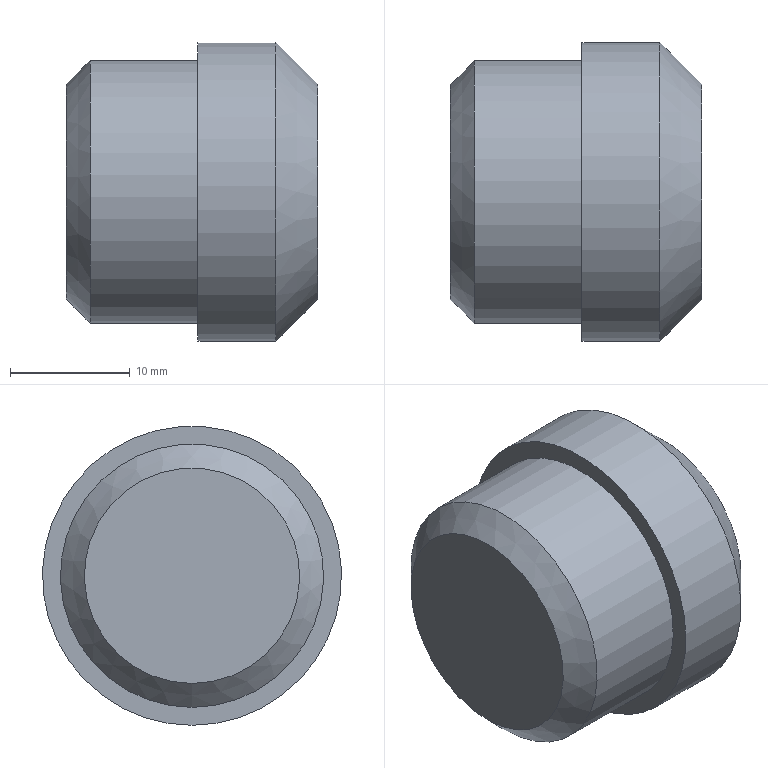Component | NX | TOP_BLOCK | 1 solid | 7 faces | box 21 x 25 x 25 mm | volume 8524 mm3 | plane 3 | cone 2 | cylinder 2 | commonest cylinder face diameters 25 x1 22 x1
STEP:
#1=CARTESIAN_POINT('',(0.,0.,0.));
#2=DIRECTION('',(0.,0.,1.));
#3=DIRECTION('',(1.,0.,0.));
#4=AXIS2_PLACEMENT_3D('',#1,#2,#3);
#5=CARTESIAN_POINT('',(95.,0.,-9.));
#6=VERTEX_POINT('',#5);
#7=CARTESIAN_POINT('',(95.,0.,0.));
#8=DIRECTION('',(1.,0.,0.));
#9=DIRECTION('',(0.,0.,-1.));
#10=AXIS2_PLACEMENT_3D('',#7,#8,#9);
#11=CIRCLE('',#10,9.);
#12=CARTESIAN_POINT('',(95.,0.,0.));
#13=DIRECTION('',(1.,0.,0.));
#14=DIRECTION('',(0.,0.,-1.));
#15=AXIS2_PLACEMENT_3D('',#12,#13,#14);
#16=PLANE('',#15);
#17=CARTESIAN_POINT('',(0.,0.));
#18=DIRECTION('',(1.,0.));
#19=AXIS2_PLACEMENT_2D('',#17,#18);
#20=CIRCLE('',#19,9.);
#21=(GEOMETRIC_REPRESENTATION_CONTEXT(2)PARAMETRIC_REPRESENTATION_CONTEXT()REPRESENTATION_CONTEXT('',''));
#22=DEFINITIONAL_REPRESENTATION('',(#20),#21);
#23=PCURVE('',#16,#22);
#24=CARTESIAN_POINT('',(95.,0.,0.));
#25=DIRECTION('',(1.,0.,0.));
#26=DIRECTION('',(0.,0.,-1.));
#27=AXIS2_PLACEMENT_3D('',#24,#25,#26);
#28=CONICAL_SURFACE('',#27,9.,0.7854);
#29=CARTESIAN_POINT('',(0.,0.));
#30=DIRECTION('',(1.,0.));
#31=VECTOR('',#30,1.);
#32=LINE('',#29,#31);
#33=(GEOMETRIC_REPRESENTATION_CONTEXT(2)PARAMETRIC_REPRESENTATION_CONTEXT()REPRESENTATION_CONTEXT('',''));
#34=DEFINITIONAL_REPRESENTATION('',(#32),#33);
#35=PCURVE('',#28,#34);
#36=SURFACE_CURVE('',#11,(#23,#35),.PCURVE_S1.);
#37=EDGE_CURVE('',#6,#6,#36,.T.);
#38=ORIENTED_EDGE('',*,*,#37,.F.);
#39=EDGE_LOOP('',(#38));
#40=FACE_BOUND('',#39,.T.);
#41=ADVANCED_FACE('',(#40),#16,.F.);
#42=CARTESIAN_POINT('',(116.,0.,-9.));
#43=VERTEX_POINT('',#42);
#44=CARTESIAN_POINT('',(116.,0.,0.));
#45=DIRECTION('',(1.,0.,0.));
#46=DIRECTION('',(0.,0.,-1.));
#47=AXIS2_PLACEMENT_3D('',#44,#45,#46);
#48=CIRCLE('',#47,9.);
#49=CARTESIAN_POINT('',(116.,0.,0.));
#50=DIRECTION('',(1.,0.,0.));
#51=DIRECTION('',(0.,0.,-1.));
#52=AXIS2_PLACEMENT_3D('',#49,#50,#51);
#53=PLANE('',#52);
#54=CARTESIAN_POINT('',(0.,0.));
#55=DIRECTION('',(1.,0.));
#56=AXIS2_PLACEMENT_2D('',#54,#55);
#57=CIRCLE('',#56,9.);
#58=(GEOMETRIC_REPRESENTATION_CONTEXT(2)PARAMETRIC_REPRESENTATION_CONTEXT()REPRESENTATION_CONTEXT('',''));
#59=DEFINITIONAL_REPRESENTATION('',(#57),#58);
#60=PCURVE('',#53,#59);
#61=CARTESIAN_POINT('',(112.5,0.,0.));
#62=DIRECTION('',(-1.,0.,0.));
#63=DIRECTION('',(0.,0.,1.));
#64=AXIS2_PLACEMENT_3D('',#61,#62,#63);
#65=CONICAL_SURFACE('',#64,12.5,0.7854);
#66=CARTESIAN_POINT('',(9.425,-3.5));
#67=DIRECTION('',(-1.,0.));
#68=VECTOR('',#67,1.);
#69=LINE('',#66,#68);
#70=(GEOMETRIC_REPRESENTATION_CONTEXT(2)PARAMETRIC_REPRESENTATION_CONTEXT()REPRESENTATION_CONTEXT('',''));
#71=DEFINITIONAL_REPRESENTATION('',(#69),#70);
#72=PCURVE('',#65,#71);
#73=SURFACE_CURVE('',#48,(#60,#72),.PCURVE_S1.);
#74=EDGE_CURVE('',#43,#43,#73,.T.);
#75=ORIENTED_EDGE('',*,*,#74,.T.);
#76=EDGE_LOOP('',(#75));
#77=FACE_BOUND('',#76,.T.);
#78=ADVANCED_FACE('',(#77),#53,.T.);
#79=ORIENTED_EDGE('',*,*,#74,.F.);
#80=CARTESIAN_POINT('',(112.5,0.,-12.5));
#81=VERTEX_POINT('',#80);
#82=CARTESIAN_POINT('',(116.,0.,-9.));
#83=CARTESIAN_POINT('',(112.5,0.,-12.5));
#84=B_SPLINE_CURVE_WITH_KNOTS('',1,(#82,#83),.UNSPECIFIED.,.F.,.F.,(2,2),(-4.95,0.),.PIECEWISE_BEZIER_KNOTS.);
#85=CARTESIAN_POINT('',(9.425,0.));
#86=DIRECTION('',(0.,1.));
#87=VECTOR('',#86,1.);
#88=LINE('',#85,#87);
#89=(GEOMETRIC_REPRESENTATION_CONTEXT(2)PARAMETRIC_REPRESENTATION_CONTEXT()REPRESENTATION_CONTEXT('',''));
#90=DEFINITIONAL_REPRESENTATION('',(#88),#89);
#91=PCURVE('',#65,#90);
#92=CARTESIAN_POINT('',(3.142,0.));
#93=DIRECTION('',(0.,1.));
#94=VECTOR('',#93,1.);
#95=LINE('',#92,#94);
#96=(GEOMETRIC_REPRESENTATION_CONTEXT(2)PARAMETRIC_REPRESENTATION_CONTEXT()REPRESENTATION_CONTEXT('',''));
#97=DEFINITIONAL_REPRESENTATION('',(#95),#96);
#98=PCURVE('',#65,#97);
#99=SEAM_CURVE('',#84,(#91,#98),.PCURVE_S1.);
#100=EDGE_CURVE('',#43,#81,#99,.T.);
#101=ORIENTED_EDGE('',*,*,#100,.T.);
#102=CARTESIAN_POINT('',(112.5,0.,0.));
#103=DIRECTION('',(1.,0.,0.));
#104=DIRECTION('',(0.,0.,-1.));
#105=AXIS2_PLACEMENT_3D('',#102,#103,#104);
#106=CIRCLE('',#105,12.5);
#107=CARTESIAN_POINT('',(9.425,0.));
#108=DIRECTION('',(-1.,0.));
#109=VECTOR('',#108,1.);
#110=LINE('',#107,#109);
#111=(GEOMETRIC_REPRESENTATION_CONTEXT(2)PARAMETRIC_REPRESENTATION_CONTEXT()REPRESENTATION_CONTEXT('',''));
#112=DEFINITIONAL_REPRESENTATION('',(#110),#111);
#113=PCURVE('',#65,#112);
#114=CARTESIAN_POINT('',(95.,0.,0.));
#115=DIRECTION('',(1.,0.,0.));
#116=DIRECTION('',(0.,0.,-1.));
#117=AXIS2_PLACEMENT_3D('',#114,#115,#116);
#118=CYLINDRICAL_SURFACE('',#117,12.5);
#119=CARTESIAN_POINT('',(0.,17.5));
#120=DIRECTION('',(1.,0.));
#121=VECTOR('',#120,1.);
#122=LINE('',#119,#121);
#123=(GEOMETRIC_REPRESENTATION_CONTEXT(2)PARAMETRIC_REPRESENTATION_CONTEXT()REPRESENTATION_CONTEXT('',''));
#124=DEFINITIONAL_REPRESENTATION('',(#122),#123);
#125=PCURVE('',#118,#124);
#126=SURFACE_CURVE('',#106,(#113,#125),.PCURVE_S1.);
#127=EDGE_CURVE('',#81,#81,#126,.T.);
#128=ORIENTED_EDGE('',*,*,#127,.T.);
#129=ORIENTED_EDGE('',*,*,#100,.F.);
#130=EDGE_LOOP('',(#79,#101,#128,#129));
#131=FACE_BOUND('',#130,.T.);
#132=ADVANCED_FACE('',(#131),#65,.T.);
#133=ORIENTED_EDGE('',*,*,#127,.F.);
#134=CARTESIAN_POINT('',(106.,0.,-12.5));
#135=VERTEX_POINT('',#134);
#136=CARTESIAN_POINT('',(106.,-0.,-12.5));
#137=CARTESIAN_POINT('',(112.5,-0.,-12.5));
#138=B_SPLINE_CURVE_WITH_KNOTS('',1,(#136,#137),.UNSPECIFIED.,.F.,.F.,(2,2),(11.,17.5),.PIECEWISE_BEZIER_KNOTS.);
#139=CARTESIAN_POINT('',(0.,0.));
#140=DIRECTION('',(0.,1.));
#141=VECTOR('',#140,1.);
#142=LINE('',#139,#141);
#143=(GEOMETRIC_REPRESENTATION_CONTEXT(2)PARAMETRIC_REPRESENTATION_CONTEXT()REPRESENTATION_CONTEXT('',''));
#144=DEFINITIONAL_REPRESENTATION('',(#142),#143);
#145=PCURVE('',#118,#144);
#146=CARTESIAN_POINT('',(6.283,0.));
#147=DIRECTION('',(0.,1.));
#148=VECTOR('',#147,1.);
#149=LINE('',#146,#148);
#150=(GEOMETRIC_REPRESENTATION_CONTEXT(2)PARAMETRIC_REPRESENTATION_CONTEXT()REPRESENTATION_CONTEXT('',''));
#151=DEFINITIONAL_REPRESENTATION('',(#149),#150);
#152=PCURVE('',#118,#151);
#153=SEAM_CURVE('',#138,(#145,#152),.PCURVE_S1.);
#154=EDGE_CURVE('',#135,#81,#153,.T.);
#155=ORIENTED_EDGE('',*,*,#154,.F.);
#156=CARTESIAN_POINT('',(106.,0.,0.));
#157=DIRECTION('',(1.,0.,0.));
#158=DIRECTION('',(0.,0.,-1.));
#159=AXIS2_PLACEMENT_3D('',#156,#157,#158);
#160=CIRCLE('',#159,12.5);
#161=CARTESIAN_POINT('',(0.,11.));
#162=DIRECTION('',(1.,0.));
#163=VECTOR('',#162,1.);
#164=LINE('',#161,#163);
#165=(GEOMETRIC_REPRESENTATION_CONTEXT(2)PARAMETRIC_REPRESENTATION_CONTEXT()REPRESENTATION_CONTEXT('',''));
#166=DEFINITIONAL_REPRESENTATION('',(#164),#165);
#167=PCURVE('',#118,#166);
#168=CARTESIAN_POINT('',(106.,11.,0.));
#169=DIRECTION('',(1.,0.,0.));
#170=DIRECTION('',(0.,0.,-1.));
#171=AXIS2_PLACEMENT_3D('',#168,#169,#170);
#172=PLANE('',#171);
#173=CARTESIAN_POINT('',(0.,-11.));
#174=DIRECTION('',(1.,0.));
#175=AXIS2_PLACEMENT_2D('',#173,#174);
#176=CIRCLE('',#175,12.5);
#177=(GEOMETRIC_REPRESENTATION_CONTEXT(2)PARAMETRIC_REPRESENTATION_CONTEXT()REPRESENTATION_CONTEXT('',''));
#178=DEFINITIONAL_REPRESENTATION('',(#176),#177);
#179=PCURVE('',#172,#178);
#180=SURFACE_CURVE('',#160,(#167,#179),.PCURVE_S1.);
#181=EDGE_CURVE('',#135,#135,#180,.T.);
#182=ORIENTED_EDGE('',*,*,#181,.T.);
#183=ORIENTED_EDGE('',*,*,#154,.T.);
#184=EDGE_LOOP('',(#133,#155,#182,#183));
#185=FACE_BOUND('',#184,.T.);
#186=ADVANCED_FACE('',(#185),#118,.T.);
#187=ORIENTED_EDGE('',*,*,#181,.F.);
#188=EDGE_LOOP('',(#187));
#189=FACE_BOUND('',#188,.T.);
#190=CARTESIAN_POINT('',(106.,0.,-11.));
#191=VERTEX_POINT('',#190);
#192=CARTESIAN_POINT('',(106.,0.,0.));
#193=DIRECTION('',(1.,0.,0.));
#194=DIRECTION('',(0.,0.,-1.));
#195=AXIS2_PLACEMENT_3D('',#192,#193,#194);
#196=CIRCLE('',#195,11.);
#197=CARTESIAN_POINT('',(0.,-11.));
#198=DIRECTION('',(1.,0.));
#199=AXIS2_PLACEMENT_2D('',#197,#198);
#200=CIRCLE('',#199,11.);
#201=(GEOMETRIC_REPRESENTATION_CONTEXT(2)PARAMETRIC_REPRESENTATION_CONTEXT()REPRESENTATION_CONTEXT('',''));
#202=DEFINITIONAL_REPRESENTATION('',(#200),#201);
#203=PCURVE('',#172,#202);
#204=CARTESIAN_POINT('',(95.,0.,0.));
#205=DIRECTION('',(1.,0.,0.));
#206=DIRECTION('',(0.,0.,-1.));
#207=AXIS2_PLACEMENT_3D('',#204,#205,#206);
#208=CYLINDRICAL_SURFACE('',#207,11.);
#209=CARTESIAN_POINT('',(0.,11.));
#210=DIRECTION('',(1.,0.));
#211=VECTOR('',#210,1.);
#212=LINE('',#209,#211);
#213=(GEOMETRIC_REPRESENTATION_CONTEXT(2)PARAMETRIC_REPRESENTATION_CONTEXT()REPRESENTATION_CONTEXT('',''));
#214=DEFINITIONAL_REPRESENTATION('',(#212),#213);
#215=PCURVE('',#208,#214);
#216=SURFACE_CURVE('',#196,(#203,#215),.PCURVE_S1.);
#217=EDGE_CURVE('',#191,#191,#216,.T.);
#218=ORIENTED_EDGE('',*,*,#217,.T.);
#219=EDGE_LOOP('',(#218));
#220=FACE_BOUND('',#219,.T.);
#221=ADVANCED_FACE('',(#189,#220),#172,.F.);
#222=ORIENTED_EDGE('',*,*,#217,.F.);
#223=CARTESIAN_POINT('',(97.,0.,-11.));
#224=VERTEX_POINT('',#223);
#225=CARTESIAN_POINT('',(97.,-0.,-11.));
#226=CARTESIAN_POINT('',(106.,-0.,-11.));
#227=B_SPLINE_CURVE_WITH_KNOTS('',1,(#225,#226),.UNSPECIFIED.,.F.,.F.,(2,2),(2.,11.),.PIECEWISE_BEZIER_KNOTS.);
#228=CARTESIAN_POINT('',(0.,0.));
#229=DIRECTION('',(0.,1.));
#230=VECTOR('',#229,1.);
#231=LINE('',#228,#230);
#232=(GEOMETRIC_REPRESENTATION_CONTEXT(2)PARAMETRIC_REPRESENTATION_CONTEXT()REPRESENTATION_CONTEXT('',''));
#233=DEFINITIONAL_REPRESENTATION('',(#231),#232);
#234=PCURVE('',#208,#233);
#235=CARTESIAN_POINT('',(6.283,0.));
#236=DIRECTION('',(0.,1.));
#237=VECTOR('',#236,1.);
#238=LINE('',#235,#237);
#239=(GEOMETRIC_REPRESENTATION_CONTEXT(2)PARAMETRIC_REPRESENTATION_CONTEXT()REPRESENTATION_CONTEXT('',''));
#240=DEFINITIONAL_REPRESENTATION('',(#238),#239);
#241=PCURVE('',#208,#240);
#242=SEAM_CURVE('',#227,(#234,#241),.PCURVE_S1.);
#243=EDGE_CURVE('',#224,#191,#242,.T.);
#244=ORIENTED_EDGE('',*,*,#243,.F.);
#245=CARTESIAN_POINT('',(97.,0.,0.));
#246=DIRECTION('',(1.,0.,0.));
#247=DIRECTION('',(0.,0.,-1.));
#248=AXIS2_PLACEMENT_3D('',#245,#246,#247);
#249=CIRCLE('',#248,11.);
#250=CARTESIAN_POINT('',(0.,2.));
#251=DIRECTION('',(1.,0.));
#252=VECTOR('',#251,1.);
#253=LINE('',#250,#252);
#254=(GEOMETRIC_REPRESENTATION_CONTEXT(2)PARAMETRIC_REPRESENTATION_CONTEXT()REPRESENTATION_CONTEXT('',''));
#255=DEFINITIONAL_REPRESENTATION('',(#253),#254);
#256=PCURVE('',#208,#255);
#257=CARTESIAN_POINT('',(0.,2.));
#258=DIRECTION('',(1.,0.));
#259=VECTOR('',#258,1.);
#260=LINE('',#257,#259);
#261=(GEOMETRIC_REPRESENTATION_CONTEXT(2)PARAMETRIC_REPRESENTATION_CONTEXT()REPRESENTATION_CONTEXT('',''));
#262=DEFINITIONAL_REPRESENTATION('',(#260),#261);
#263=PCURVE('',#28,#262);
#264=SURFACE_CURVE('',#249,(#256,#263),.PCURVE_S1.);
#265=EDGE_CURVE('',#224,#224,#264,.T.);
#266=ORIENTED_EDGE('',*,*,#265,.T.);
#267=ORIENTED_EDGE('',*,*,#243,.T.);
#268=EDGE_LOOP('',(#222,#244,#266,#267));
#269=FACE_BOUND('',#268,.T.);
#270=ADVANCED_FACE('',(#269),#208,.T.);
#271=ORIENTED_EDGE('',*,*,#265,.F.);
#272=CARTESIAN_POINT('',(95.,-0.,-9.));
#273=CARTESIAN_POINT('',(97.,-0.,-11.));
#274=B_SPLINE_CURVE_WITH_KNOTS('',1,(#272,#273),.UNSPECIFIED.,.F.,.F.,(2,2),(0.,2.828),.PIECEWISE_BEZIER_KNOTS.);
#275=CARTESIAN_POINT('',(0.,0.));
#276=DIRECTION('',(0.,1.));
#277=VECTOR('',#276,1.);
#278=LINE('',#275,#277);
#279=(GEOMETRIC_REPRESENTATION_CONTEXT(2)PARAMETRIC_REPRESENTATION_CONTEXT()REPRESENTATION_CONTEXT('',''));
#280=DEFINITIONAL_REPRESENTATION('',(#278),#279);
#281=PCURVE('',#28,#280);
#282=CARTESIAN_POINT('',(6.283,0.));
#283=DIRECTION('',(0.,1.));
#284=VECTOR('',#283,1.);
#285=LINE('',#282,#284);
#286=(GEOMETRIC_REPRESENTATION_CONTEXT(2)PARAMETRIC_REPRESENTATION_CONTEXT()REPRESENTATION_CONTEXT('',''));
#287=DEFINITIONAL_REPRESENTATION('',(#285),#286);
#288=PCURVE('',#28,#287);
#289=SEAM_CURVE('',#274,(#281,#288),.PCURVE_S1.);
#290=EDGE_CURVE('',#6,#224,#289,.T.);
#291=ORIENTED_EDGE('',*,*,#290,.F.);
#292=ORIENTED_EDGE('',*,*,#37,.T.);
#293=ORIENTED_EDGE('',*,*,#290,.T.);
#294=EDGE_LOOP('',(#271,#291,#292,#293));
#295=FACE_BOUND('',#294,.T.);
#296=ADVANCED_FACE('',(#295),#28,.T.);
#297=CLOSED_SHELL('',(#41,#78,#132,#186,#221,#270,#296));
#298=MANIFOLD_SOLID_BREP('',#297);
#299=(LENGTH_UNIT()NAMED_UNIT(*)SI_UNIT(.MILLI.,.METRE.));
#300=UNCERTAINTY_MEASURE_WITH_UNIT(LENGTH_MEASURE(0.00001),#299,'','');
#301=(NAMED_UNIT(*)PLANE_ANGLE_UNIT()SI_UNIT($,.RADIAN.));
#302=(NAMED_UNIT(*)SI_UNIT($,.STERADIAN.)SOLID_ANGLE_UNIT());
#303=(GEOMETRIC_REPRESENTATION_CONTEXT(3)GLOBAL_UNCERTAINTY_ASSIGNED_CONTEXT((#300))GLOBAL_UNIT_ASSIGNED_CONTEXT((#299,#301,#302))REPRESENTATION_CONTEXT('',''));
#304=ADVANCED_BREP_SHAPE_REPRESENTATION('',(#4,#298),#303);